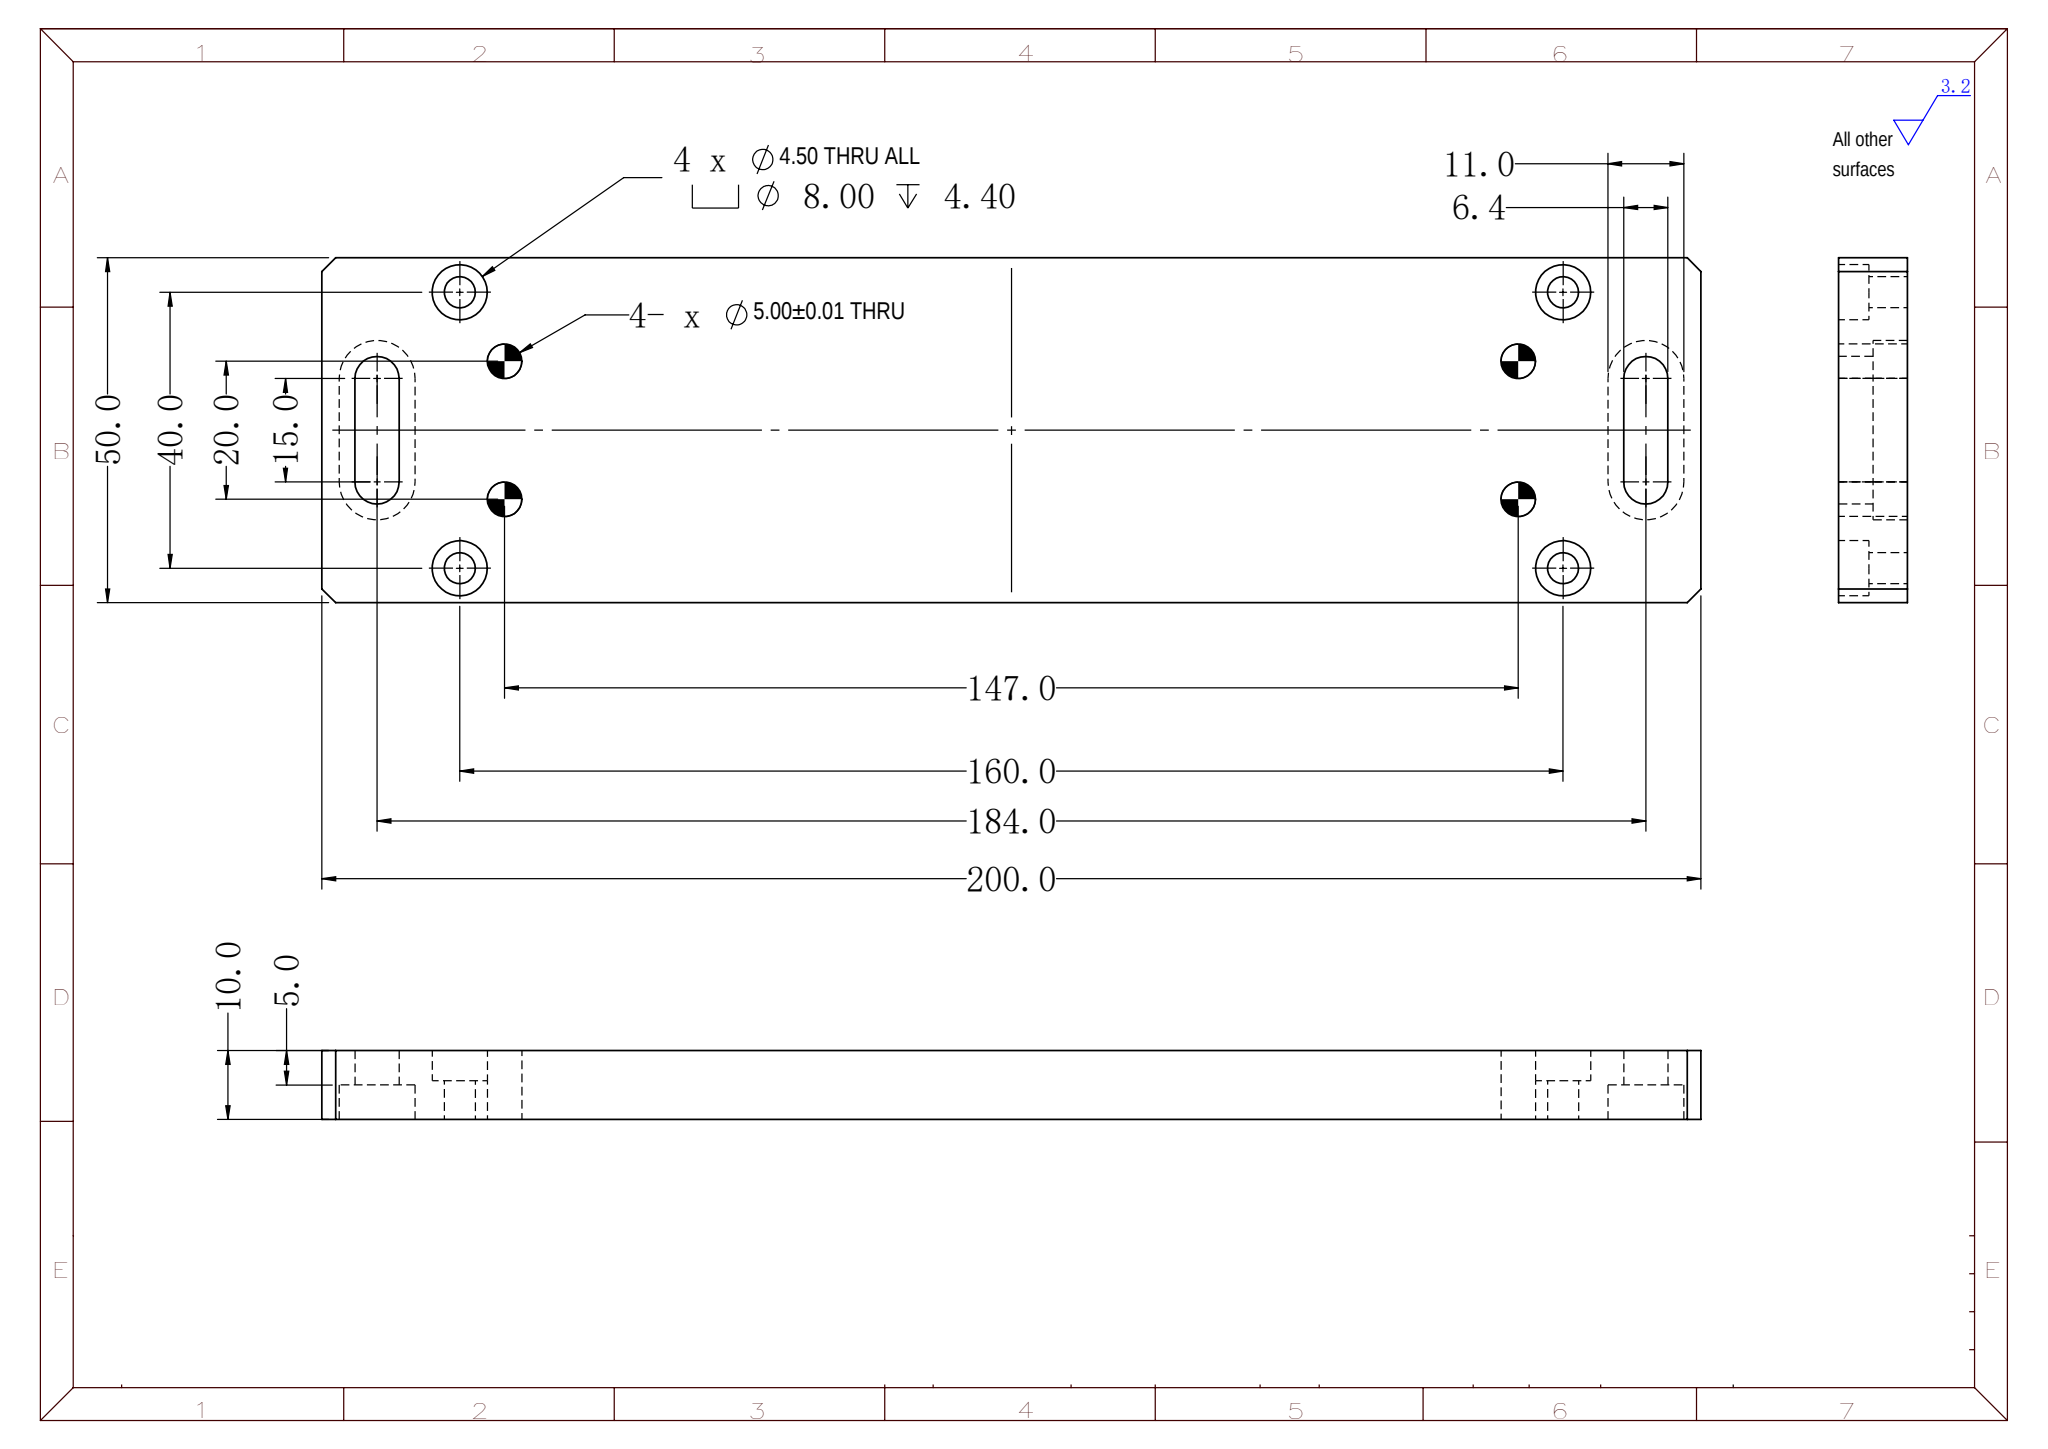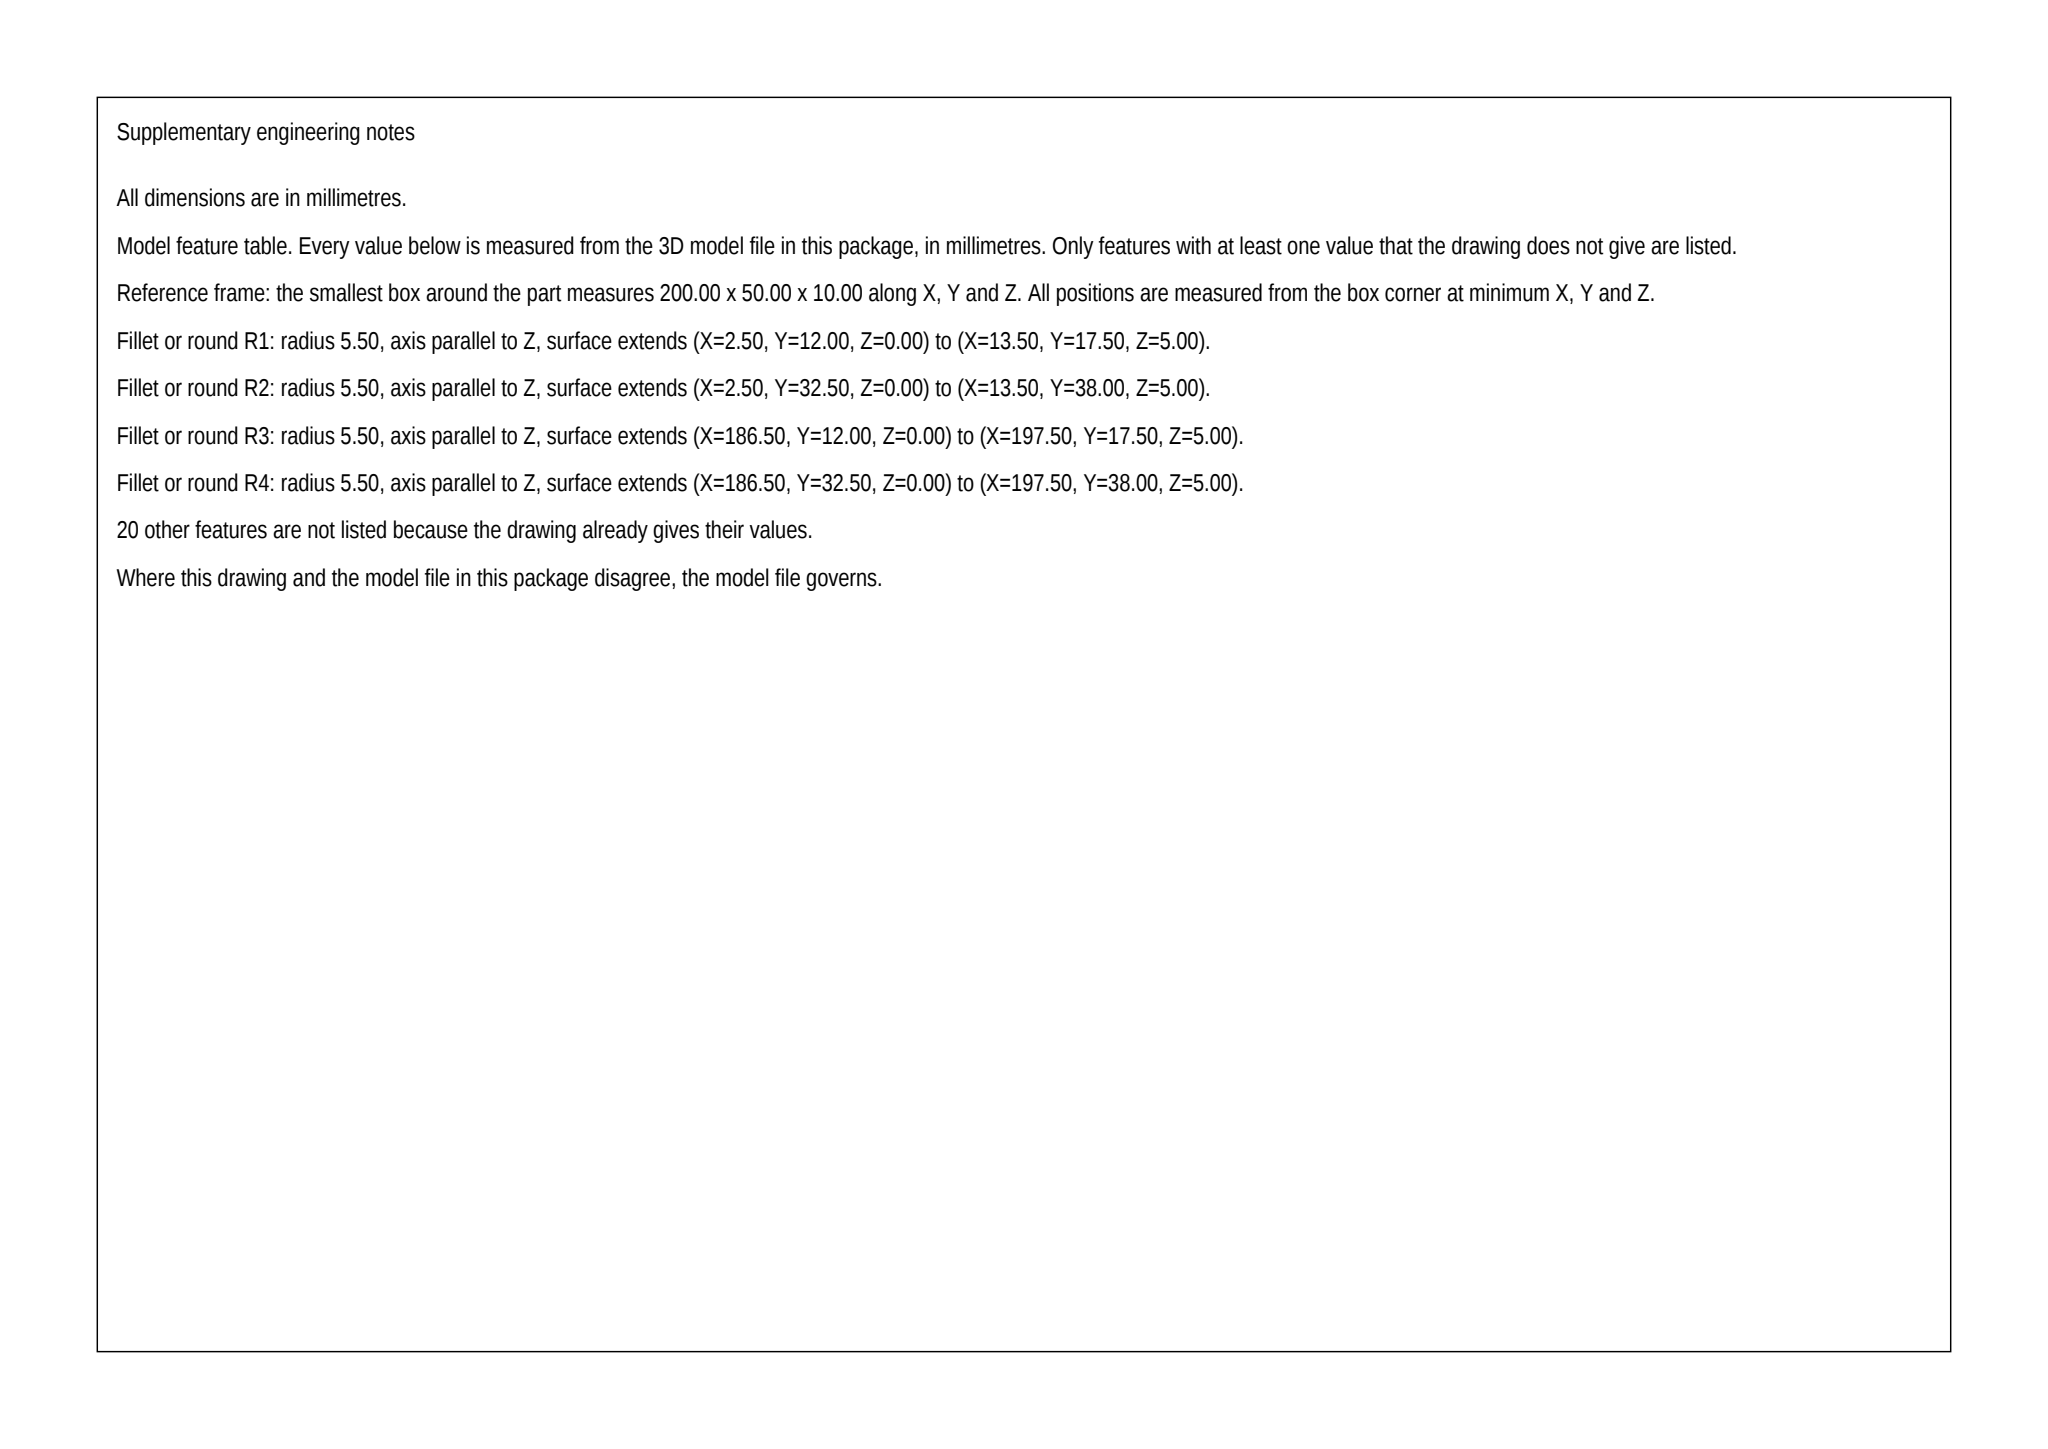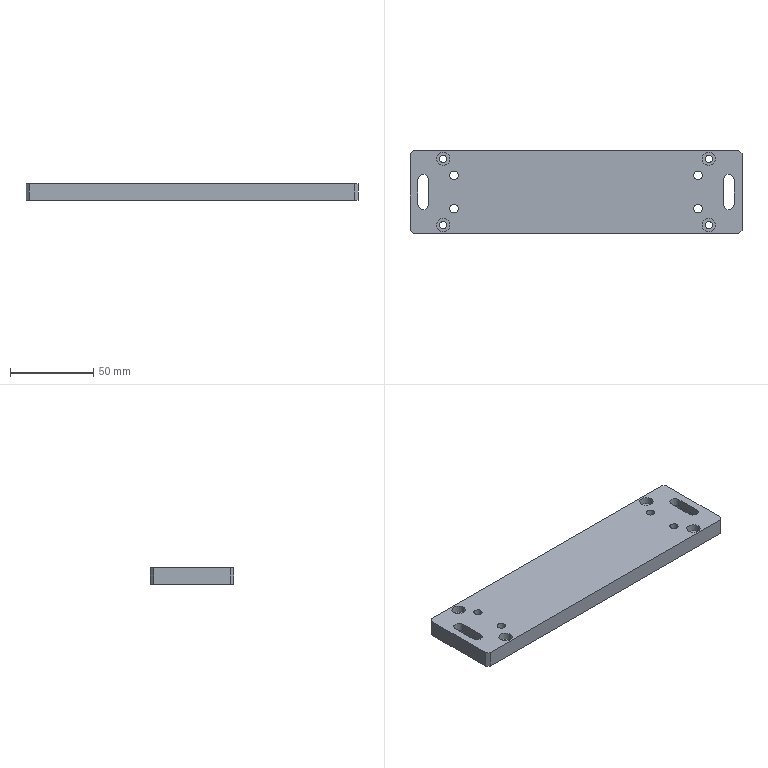Part | SolidWorks | mm | 1 solid | 56 faces | box 200 x 50 x 10 mm | volume 94012 mm3 | cylinder 32 | plane 24 | commonest cylinder face diameters 5 x8 8 x8 4.5 x8 6.4 x4 11 x4
build123d program:
from build123d import *

# Parameters (mm, degrees)
SKETCH1_W                                       = 200
SKETCH1_H                                       = 50
BOSS_EXTRUDE1_DEPTH                             = 10
CUT_EXTRUDE1_DEPTH                              = 104.562
CUT_EXTRUDE2_DEPTH                              = 5
M4_HEX_SOCKET_HEAD_CAP_SCREW_CBORE1_D           = 4.5
M4_HEX_SOCKET_HEAD_CAP_SCREW_CBORE1_CBORE_D     = 8
M4_HEX_SOCKET_HEAD_CAP_SCREW_CBORE1_CBORE_DEPTH = 4.4
CHAMFER1_SIZE                                   = 2
SIZE_MM_DOWEL_PIN_HOLE1_D                       = 5


with BuildPart() as part:
    # Sketch1 → Boss-Extrude1 (new body)
    with BuildSketch(Plane.XY):
        Rectangle(SKETCH1_W, SKETCH1_H)
    extrude(amount=BOSS_EXTRUDE1_DEPTH)

    # Sketch6 → Cut-Extrude1 (cut, through all)
    with BuildSketch(Plane(origin=(0, 0, 0), x_dir=(-1, 0, 0), z_dir=(0, 0, -1))):
        with BuildLine():
            Line((95.2, 7.5), (95.2, -7.5))
            ThreePointArc((95.2, -7.5), (92, -10.7), (88.8, -7.5))
            Line((88.8, -7.5), (88.8, 7.5))
            ThreePointArc((88.8, 7.5), (92, 10.7), (95.2, 7.5))
        make_face()
    cut_extrude1 = extrude(amount=-CUT_EXTRUDE1_DEPTH, mode=Mode.SUBTRACT)

    # Sketch7 → Cut-Extrude2 (cut)
    with BuildSketch(Plane(origin=(0, 0, 0), x_dir=(-1, 0, 0), z_dir=(0, 0, -1))):
        with BuildLine():
            Line((97.5, 7.5), (97.5, -7.5))
            ThreePointArc((97.5, -7.5), (92, -13), (86.5, -7.5))
            Line((86.5, -7.5), (86.5, 7.5))
            ThreePointArc((86.5, 7.5), (92, 13), (97.5, 7.5))
        make_face()
    cut_extrude2 = extrude(amount=-CUT_EXTRUDE2_DEPTH, mode=Mode.SUBTRACT)

    # M4 Hex Socket Head Cap Screw CBORE1 (through all)
    with Locations(Plane(origin=(-80, 20, 10), x_dir=(1, 0, 0), z_dir=(0, 0, 1))):
        with Locations((0, 0), (0, -40)):
            m4_hex_socket_head_cap_screw_cbore1 = CounterBoreHole(M4_HEX_SOCKET_HEAD_CAP_SCREW_CBORE1_D / 2, M4_HEX_SOCKET_HEAD_CAP_SCREW_CBORE1_CBORE_D / 2, M4_HEX_SOCKET_HEAD_CAP_SCREW_CBORE1_CBORE_DEPTH)

    # Mirror1: Cut-Extrude1, Cut-Extrude2, M4 Hex Socket Head Cap Screw CBORE1 across plane
    add(cut_extrude1.mirror(Plane(origin=(0, 0, 0), x_dir=(0, 0, 1), z_dir=(1, 0, 0))), mode=Mode.SUBTRACT)
    add(cut_extrude2.mirror(Plane(origin=(0, 0, 0), x_dir=(0, 0, 1), z_dir=(1, 0, 0))), mode=Mode.SUBTRACT)
    add(m4_hex_socket_head_cap_screw_cbore1.mirror(Plane(origin=(0, 0, 0), x_dir=(0, 0, 1), z_dir=(1, 0, 0))), mode=Mode.SUBTRACT)

    # Chamfer1
    chamfer1_edges = [part.edges().sort_by_distance(p)[0] for p in [
        (100, -25, 5),
        (-100, -25, 5),
        (-100, 25, 5),
        (100, 25, 5),
    ]]
    chamfer(chamfer1_edges, length=CHAMFER1_SIZE)

    # Size mm Dowel Pin Hole1 (through all)
    with Locations(Plane(origin=(73.5, 10, 0), x_dir=(-1, 0, 0), z_dir=(0, 0, -1))):
        with Locations((0, 0), (0, -20)):
            size_mm_dowel_pin_hole1 = Hole(SIZE_MM_DOWEL_PIN_HOLE1_D / 2)

    # Mirror2: Size mm Dowel Pin Hole1 across plane
    add(size_mm_dowel_pin_hole1.mirror(Plane(origin=(0, 0, 0), x_dir=(0, 0, 1), z_dir=(1, 0, 0))), mode=Mode.SUBTRACT)


solid = part.part